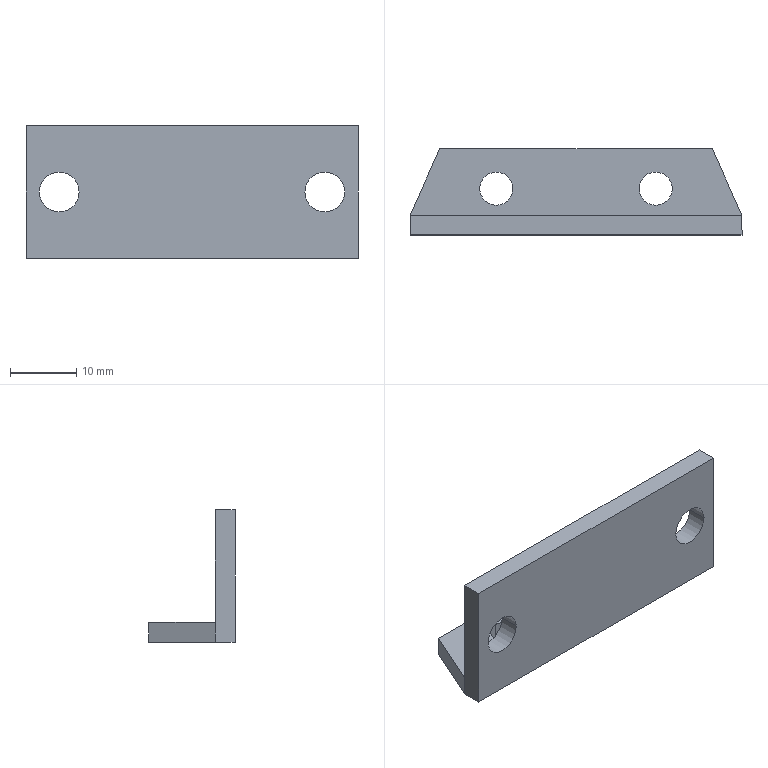Component | SolidWorks | Stand-2 | 1 solid | 18 faces | box 50 x 13 x 20 mm | volume 4078 mm3 | plane 10 | cylinder 8 | commonest cylinder face diameters 5 x4 6 x4
build123d program:
from build123d import *

# Parameters (mm, degrees)
SKETCH1_W      = 50
SKETCH1_H      = 20
SKETCH1_R      = 3
EXTRUDE1_DEPTH = 3
SKETCH2_R      = 2.5
EXTRUDE2_DEPTH = 3


with BuildPart() as part:
    # Sketch1 → Extrude1 (new body)
    with BuildSketch(Plane.XY):
        with Locations((-4.582, -13.446)):
            Rectangle(SKETCH1_W, SKETCH1_H)
        with Locations((-24.582, -13.446)):
            Circle(SKETCH1_R, mode=Mode.SUBTRACT)
        with Locations((15.418, -13.446)):
            Circle(SKETCH1_R, mode=Mode.SUBTRACT)
    extrude(amount=EXTRUDE1_DEPTH)

    # Sketch2 → Extrude2 (add)
    with BuildSketch(Plane.XZ.offset(23.446)):
        Polygon((-29.582, 3), (-25.108, 13), (15.944, 13), (20.418, 3), align=None)
        with Locations(Location((-16.582, 7, 0), (0, 0, 270))):
            Circle(SKETCH2_R, mode=Mode.SUBTRACT)
        with Locations(Location((7.418, 7, 0), (0, 0, 90))):
            Circle(SKETCH2_R, mode=Mode.SUBTRACT)
    extrude(amount=-EXTRUDE2_DEPTH)


solid = part.part

# Placed as in the assembly
solid = solid.moved(Location((1.543, -20.646, 12.946), (-90, 0, 180)))
STEP:
#1=COLOUR_RGB('',0.7922,0.8196,0.9333);
#2=FILL_AREA_STYLE_COLOUR('',#1);
#3=FILL_AREA_STYLE('',(#2));
#4=SURFACE_STYLE_FILL_AREA(#3);
#5=SURFACE_SIDE_STYLE('',(#4));
#6=SURFACE_STYLE_USAGE(.BOTH.,#5);
#7=PRESENTATION_STYLE_ASSIGNMENT((#6));
#8=CARTESIAN_POINT('',(-0.2313,-0.4388,-0.2953));
#9=VERTEX_POINT('',#8);
#10=CARTESIAN_POINT('',(-0.2313,-0.6357,-0.2953));
#11=VERTEX_POINT('',#10);
#12=CARTESIAN_POINT('',(-0.2313,-0.5373,-0.2953));
#13=DIRECTION('',(0.,0.,-1.));
#14=DIRECTION('',(-0.,1.,0.));
#15=AXIS2_PLACEMENT_3D('',#12,#13,#14);
#16=CIRCLE('',#15,0.09843);
#17=EDGE_CURVE('',#9,#11,#16,.T.);
#18=ORIENTED_EDGE('',*,*,#17,.F.);
#19=CARTESIAN_POINT('',(-0.2313,-0.4388,-0.4134));
#20=VERTEX_POINT('',#19);
#21=CARTESIAN_POINT('',(-0.2313,-0.4388,-0.2953));
#22=DIRECTION('',(0.,0.,-1.));
#23=VECTOR('',#22,39.37);
#24=LINE('',#21,#23);
#25=EDGE_CURVE('',#9,#20,#24,.T.);
#26=ORIENTED_EDGE('',*,*,#25,.T.);
#27=CARTESIAN_POINT('',(-0.2313,-0.6357,-0.4134));
#28=VERTEX_POINT('',#27);
#29=CARTESIAN_POINT('',(-0.2313,-0.5373,-0.4134));
#30=DIRECTION('',(0.,0.,-1.));
#31=DIRECTION('',(-0.,1.,0.));
#32=AXIS2_PLACEMENT_3D('',#29,#30,#31);
#33=CIRCLE('',#32,0.09843);
#34=EDGE_CURVE('',#20,#28,#33,.T.);
#35=ORIENTED_EDGE('',*,*,#34,.T.);
#36=CARTESIAN_POINT('',(-0.2313,-0.6357,-0.2953));
#37=DIRECTION('',(0.,0.,-1.));
#38=VECTOR('',#37,39.37);
#39=LINE('',#36,#38);
#40=EDGE_CURVE('',#11,#28,#39,.T.);
#41=ORIENTED_EDGE('',*,*,#40,.F.);
#42=EDGE_LOOP('',(#18,#26,#35,#41));
#43=FACE_OUTER_BOUND('',#42,.T.);
#44=CARTESIAN_POINT('',(-0.2313,-0.5373,-0.2953));
#45=DIRECTION('',(0.,0.,-1.));
#46=DIRECTION('',(0.,-1.,0.));
#47=AXIS2_PLACEMENT_3D('',#44,#45,#46);
#48=CYLINDRICAL_SURFACE('',#47,0.09843);
#49=ADVANCED_FACE('',(#43),#48,.F.);
#50=CARTESIAN_POINT('',(0.7136,-0.4388,-0.2953));
#51=VERTEX_POINT('',#50);
#52=CARTESIAN_POINT('',(0.7136,-0.6357,-0.2953));
#53=VERTEX_POINT('',#52);
#54=CARTESIAN_POINT('',(0.7136,-0.5373,-0.2953));
#55=DIRECTION('',(0.,0.,-1.));
#56=DIRECTION('',(0.,-1.,0.));
#57=AXIS2_PLACEMENT_3D('',#54,#55,#56);
#58=CIRCLE('',#57,0.09843);
#59=EDGE_CURVE('',#51,#53,#58,.T.);
#60=ORIENTED_EDGE('',*,*,#59,.F.);
#61=CARTESIAN_POINT('',(0.7136,-0.4388,-0.4134));
#62=VERTEX_POINT('',#61);
#63=CARTESIAN_POINT('',(0.7136,-0.4388,-0.2953));
#64=DIRECTION('',(0.,0.,-1.));
#65=VECTOR('',#64,39.37);
#66=LINE('',#63,#65);
#67=EDGE_CURVE('',#51,#62,#66,.T.);
#68=ORIENTED_EDGE('',*,*,#67,.T.);
#69=CARTESIAN_POINT('',(0.7136,-0.6357,-0.4134));
#70=VERTEX_POINT('',#69);
#71=CARTESIAN_POINT('',(0.7136,-0.5373,-0.4134));
#72=DIRECTION('',(0.,0.,-1.));
#73=DIRECTION('',(0.,-1.,0.));
#74=AXIS2_PLACEMENT_3D('',#71,#72,#73);
#75=CIRCLE('',#74,0.09843);
#76=EDGE_CURVE('',#62,#70,#75,.T.);
#77=ORIENTED_EDGE('',*,*,#76,.T.);
#78=CARTESIAN_POINT('',(0.7136,-0.6357,-0.2953));
#79=DIRECTION('',(0.,0.,-1.));
#80=VECTOR('',#79,39.37);
#81=LINE('',#78,#80);
#82=EDGE_CURVE('',#53,#70,#81,.T.);
#83=ORIENTED_EDGE('',*,*,#82,.F.);
#84=EDGE_LOOP('',(#60,#68,#77,#83));
#85=FACE_OUTER_BOUND('',#84,.T.);
#86=CARTESIAN_POINT('',(0.7136,-0.5373,-0.2953));
#87=DIRECTION('',(0.,0.,-1.));
#88=DIRECTION('',(0.,-1.,0.));
#89=AXIS2_PLACEMENT_3D('',#86,#87,#88);
#90=CYLINDRICAL_SURFACE('',#89,0.09843);
#91=ADVANCED_FACE('',(#85),#90,.F.);
#92=CARTESIAN_POINT('',(-0.4282,-0.6947,-0.01969));
#93=VERTEX_POINT('',#92);
#94=CARTESIAN_POINT('',(-0.6644,-0.6947,-0.01969));
#95=VERTEX_POINT('',#94);
#96=CARTESIAN_POINT('',(-0.5463,-0.6947,-0.01969));
#97=DIRECTION('',(-0.,1.,0.));
#98=DIRECTION('',(-1.,-0.,-0.));
#99=AXIS2_PLACEMENT_3D('',#96,#97,#98);
#100=CIRCLE('',#99,0.1181);
#101=EDGE_CURVE('',#93,#95,#100,.T.);
#102=ORIENTED_EDGE('',*,*,#101,.T.);
#103=CARTESIAN_POINT('',(-0.6644,-0.8129,-0.01969));
#104=VERTEX_POINT('',#103);
#105=CARTESIAN_POINT('',(-0.6644,-0.6947,-0.01969));
#106=DIRECTION('',(0.,-1.,-0.));
#107=VECTOR('',#106,39.37);
#108=LINE('',#105,#107);
#109=EDGE_CURVE('',#95,#104,#108,.T.);
#110=ORIENTED_EDGE('',*,*,#109,.T.);
#111=CARTESIAN_POINT('',(-0.4282,-0.8129,-0.01969));
#112=VERTEX_POINT('',#111);
#113=CARTESIAN_POINT('',(-0.5463,-0.8129,-0.01969));
#114=DIRECTION('',(-0.,1.,0.));
#115=DIRECTION('',(-1.,-0.,-0.));
#116=AXIS2_PLACEMENT_3D('',#113,#114,#115);
#117=CIRCLE('',#116,0.1181);
#118=EDGE_CURVE('',#112,#104,#117,.T.);
#119=ORIENTED_EDGE('',*,*,#118,.F.);
#120=CARTESIAN_POINT('',(-0.4282,-0.6947,-0.01969));
#121=DIRECTION('',(0.,-1.,-0.));
#122=VECTOR('',#121,39.37);
#123=LINE('',#120,#122);
#124=EDGE_CURVE('',#93,#112,#123,.T.);
#125=ORIENTED_EDGE('',*,*,#124,.F.);
#126=EDGE_LOOP('',(#102,#110,#119,#125));
#127=FACE_OUTER_BOUND('',#126,.T.);
#128=CARTESIAN_POINT('',(-0.5463,-0.6947,-0.01969));
#129=DIRECTION('',(0.,-1.,-0.));
#130=DIRECTION('',(1.,0.,0.));
#131=AXIS2_PLACEMENT_3D('',#128,#129,#130);
#132=CYLINDRICAL_SURFACE('',#131,0.1181);
#133=ADVANCED_FACE('',(#127),#132,.F.);
#134=CARTESIAN_POINT('',(1.147,-0.6947,-0.01969));
#135=VERTEX_POINT('',#134);
#136=CARTESIAN_POINT('',(0.9104,-0.6947,-0.01969));
#137=VERTEX_POINT('',#136);
#138=CARTESIAN_POINT('',(1.029,-0.6947,-0.01969));
#139=DIRECTION('',(-0.,1.,0.));
#140=DIRECTION('',(-1.,-0.,-0.));
#141=AXIS2_PLACEMENT_3D('',#138,#139,#140);
#142=CIRCLE('',#141,0.1181);
#143=EDGE_CURVE('',#135,#137,#142,.T.);
#144=ORIENTED_EDGE('',*,*,#143,.T.);
#145=CARTESIAN_POINT('',(0.9104,-0.8129,-0.01969));
#146=VERTEX_POINT('',#145);
#147=CARTESIAN_POINT('',(0.9104,-0.6947,-0.01969));
#148=DIRECTION('',(0.,-1.,-0.));
#149=VECTOR('',#148,39.37);
#150=LINE('',#147,#149);
#151=EDGE_CURVE('',#137,#146,#150,.T.);
#152=ORIENTED_EDGE('',*,*,#151,.T.);
#153=CARTESIAN_POINT('',(1.147,-0.8129,-0.01969));
#154=VERTEX_POINT('',#153);
#155=CARTESIAN_POINT('',(1.029,-0.8129,-0.01969));
#156=DIRECTION('',(-0.,1.,0.));
#157=DIRECTION('',(-1.,-0.,-0.));
#158=AXIS2_PLACEMENT_3D('',#155,#156,#157);
#159=CIRCLE('',#158,0.1181);
#160=EDGE_CURVE('',#154,#146,#159,.T.);
#161=ORIENTED_EDGE('',*,*,#160,.F.);
#162=CARTESIAN_POINT('',(1.147,-0.6947,-0.01969));
#163=DIRECTION('',(0.,-1.,-0.));
#164=VECTOR('',#163,39.37);
#165=LINE('',#162,#164);
#166=EDGE_CURVE('',#135,#154,#165,.T.);
#167=ORIENTED_EDGE('',*,*,#166,.F.);
#168=EDGE_LOOP('',(#144,#152,#161,#167));
#169=FACE_OUTER_BOUND('',#168,.T.);
#170=CARTESIAN_POINT('',(1.029,-0.6947,-0.01969));
#171=DIRECTION('',(0.,-1.,-0.));
#172=DIRECTION('',(1.,0.,0.));
#173=AXIS2_PLACEMENT_3D('',#170,#171,#172);
#174=CYLINDRICAL_SURFACE('',#173,0.1181);
#175=ADVANCED_FACE('',(#169),#174,.F.);
#176=ORIENTED_EDGE('',*,*,#101,.F.);
#177=CARTESIAN_POINT('',(-0.5463,-0.6947,-0.01969));
#178=DIRECTION('',(-0.,1.,0.));
#179=DIRECTION('',(-1.,-0.,-0.));
#180=AXIS2_PLACEMENT_3D('',#177,#178,#179);
#181=CIRCLE('',#180,0.1181);
#182=EDGE_CURVE('',#95,#93,#181,.T.);
#183=ORIENTED_EDGE('',*,*,#182,.F.);
#184=EDGE_LOOP('',(#176,#183));
#185=FACE_BOUND('',#184,.T.);
#186=ORIENTED_EDGE('',*,*,#143,.F.);
#187=CARTESIAN_POINT('',(1.029,-0.6947,-0.01969));
#188=DIRECTION('',(-0.,1.,0.));
#189=DIRECTION('',(-1.,-0.,-0.));
#190=AXIS2_PLACEMENT_3D('',#187,#188,#189);
#191=CIRCLE('',#190,0.1181);
#192=EDGE_CURVE('',#137,#135,#191,.T.);
#193=ORIENTED_EDGE('',*,*,#192,.F.);
#194=EDGE_LOOP('',(#186,#193));
#195=FACE_BOUND('',#194,.T.);
#196=CARTESIAN_POINT('',(1.225,-0.6947,0.374));
#197=VERTEX_POINT('',#196);
#198=CARTESIAN_POINT('',(1.225,-0.6947,-0.2953));
#199=VERTEX_POINT('',#198);
#200=CARTESIAN_POINT('',(1.225,-0.6947,0.374));
#201=DIRECTION('',(0.,0.,-1.));
#202=VECTOR('',#201,39.37);
#203=LINE('',#200,#202);
#204=EDGE_CURVE('',#197,#199,#203,.T.);
#205=ORIENTED_EDGE('',*,*,#204,.T.);
#206=CARTESIAN_POINT('',(-0.7431,-0.6947,-0.2953));
#207=VERTEX_POINT('',#206);
#208=CARTESIAN_POINT('',(1.225,-0.6947,-0.2953));
#209=DIRECTION('',(-1.,-0.,-0.));
#210=VECTOR('',#209,39.37);
#211=LINE('',#208,#210);
#212=EDGE_CURVE('',#199,#207,#211,.T.);
#213=ORIENTED_EDGE('',*,*,#212,.T.);
#214=CARTESIAN_POINT('',(-0.7431,-0.6947,0.374));
#215=VERTEX_POINT('',#214);
#216=CARTESIAN_POINT('',(-0.7431,-0.6947,0.374));
#217=DIRECTION('',(0.,-0.,1.));
#218=VECTOR('',#217,39.37);
#219=LINE('',#216,#218);
#220=EDGE_CURVE('',#207,#215,#219,.T.);
#221=ORIENTED_EDGE('',*,*,#220,.T.);
#222=CARTESIAN_POINT('',(1.225,-0.6947,0.374));
#223=DIRECTION('',(1.,0.,0.));
#224=VECTOR('',#223,39.37);
#225=LINE('',#222,#224);
#226=EDGE_CURVE('',#215,#197,#225,.T.);
#227=ORIENTED_EDGE('',*,*,#226,.T.);
#228=EDGE_LOOP('',(#205,#213,#221,#227));
#229=FACE_OUTER_BOUND('',#228,.T.);
#230=CARTESIAN_POINT('',(1.225,-0.6947,-0.4134));
#231=DIRECTION('',(-0.,1.,0.));
#232=DIRECTION('',(-1.,-0.,-0.));
#233=AXIS2_PLACEMENT_3D('',#230,#231,#232);
#234=PLANE('',#233);
#235=ADVANCED_FACE('',(#185,#195,#229),#234,.T.);
#236=ORIENTED_EDGE('',*,*,#160,.T.);
#237=CARTESIAN_POINT('',(1.029,-0.8129,-0.01969));
#238=DIRECTION('',(-0.,1.,0.));
#239=DIRECTION('',(-1.,-0.,-0.));
#240=AXIS2_PLACEMENT_3D('',#237,#238,#239);
#241=CIRCLE('',#240,0.1181);
#242=EDGE_CURVE('',#146,#154,#241,.T.);
#243=ORIENTED_EDGE('',*,*,#242,.T.);
#244=EDGE_LOOP('',(#236,#243));
#245=FACE_BOUND('',#244,.T.);
#246=CARTESIAN_POINT('',(1.225,-0.8129,0.374));
#247=VERTEX_POINT('',#246);
#248=CARTESIAN_POINT('',(1.225,-0.8129,-0.4134));
#249=VERTEX_POINT('',#248);
#250=CARTESIAN_POINT('',(1.225,-0.8129,0.374));
#251=DIRECTION('',(0.,0.,-1.));
#252=VECTOR('',#251,39.37);
#253=LINE('',#250,#252);
#254=EDGE_CURVE('',#247,#249,#253,.T.);
#255=ORIENTED_EDGE('',*,*,#254,.F.);
#256=CARTESIAN_POINT('',(-0.7431,-0.8129,0.374));
#257=VERTEX_POINT('',#256);
#258=CARTESIAN_POINT('',(1.225,-0.8129,0.374));
#259=DIRECTION('',(1.,0.,0.));
#260=VECTOR('',#259,39.37);
#261=LINE('',#258,#260);
#262=EDGE_CURVE('',#257,#247,#261,.T.);
#263=ORIENTED_EDGE('',*,*,#262,.F.);
#264=CARTESIAN_POINT('',(-0.7431,-0.8129,-0.4134));
#265=VERTEX_POINT('',#264);
#266=CARTESIAN_POINT('',(-0.7431,-0.8129,0.374));
#267=DIRECTION('',(0.,-0.,1.));
#268=VECTOR('',#267,39.37);
#269=LINE('',#266,#268);
#270=EDGE_CURVE('',#265,#257,#269,.T.);
#271=ORIENTED_EDGE('',*,*,#270,.F.);
#272=CARTESIAN_POINT('',(1.225,-0.8129,-0.4134));
#273=DIRECTION('',(-1.,-0.,-0.));
#274=VECTOR('',#273,39.37);
#275=LINE('',#272,#274);
#276=EDGE_CURVE('',#249,#265,#275,.T.);
#277=ORIENTED_EDGE('',*,*,#276,.F.);
#278=EDGE_LOOP('',(#255,#263,#271,#277));
#279=FACE_OUTER_BOUND('',#278,.T.);
#280=ORIENTED_EDGE('',*,*,#118,.T.);
#281=CARTESIAN_POINT('',(-0.5463,-0.8129,-0.01969));
#282=DIRECTION('',(-0.,1.,0.));
#283=DIRECTION('',(-1.,-0.,-0.));
#284=AXIS2_PLACEMENT_3D('',#281,#282,#283);
#285=CIRCLE('',#284,0.1181);
#286=EDGE_CURVE('',#104,#112,#285,.T.);
#287=ORIENTED_EDGE('',*,*,#286,.T.);
#288=EDGE_LOOP('',(#280,#287));
#289=FACE_BOUND('',#288,.T.);
#290=CARTESIAN_POINT('',(1.225,-0.8129,-0.4134));
#291=DIRECTION('',(-0.,1.,0.));
#292=DIRECTION('',(-1.,-0.,-0.));
#293=AXIS2_PLACEMENT_3D('',#290,#291,#292);
#294=PLANE('',#293);
#295=ADVANCED_FACE('',(#245,#279,#289),#294,.F.);
#296=ORIENTED_EDGE('',*,*,#254,.T.);
#297=CARTESIAN_POINT('',(1.225,-0.6947,-0.4134));
#298=VERTEX_POINT('',#297);
#299=CARTESIAN_POINT('',(1.225,-0.6947,-0.4134));
#300=DIRECTION('',(0.,-1.,-0.));
#301=VECTOR('',#300,39.37);
#302=LINE('',#299,#301);
#303=EDGE_CURVE('',#298,#249,#302,.T.);
#304=ORIENTED_EDGE('',*,*,#303,.F.);
#305=CARTESIAN_POINT('',(1.225,-0.6947,-0.2953));
#306=DIRECTION('',(0.,0.,-1.));
#307=VECTOR('',#306,39.37);
#308=LINE('',#305,#307);
#309=EDGE_CURVE('',#199,#298,#308,.T.);
#310=ORIENTED_EDGE('',*,*,#309,.F.);
#311=ORIENTED_EDGE('',*,*,#204,.F.);
#312=CARTESIAN_POINT('',(1.225,-0.6947,0.374));
#313=DIRECTION('',(0.,-1.,-0.));
#314=VECTOR('',#313,39.37);
#315=LINE('',#312,#314);
#316=EDGE_CURVE('',#197,#247,#315,.T.);
#317=ORIENTED_EDGE('',*,*,#316,.T.);
#318=EDGE_LOOP('',(#296,#304,#310,#311,#317));
#319=FACE_OUTER_BOUND('',#318,.T.);
#320=CARTESIAN_POINT('',(1.225,-0.6947,0.374));
#321=DIRECTION('',(-1.,-0.,-0.));
#322=DIRECTION('',(0.,-1.,-0.));
#323=AXIS2_PLACEMENT_3D('',#320,#321,#322);
#324=PLANE('',#323);
#325=ADVANCED_FACE('',(#319),#324,.F.);
#326=ORIENTED_EDGE('',*,*,#276,.T.);
#327=CARTESIAN_POINT('',(-0.7431,-0.6947,-0.4134));
#328=VERTEX_POINT('',#327);
#329=CARTESIAN_POINT('',(-0.7431,-0.6947,-0.4134));
#330=DIRECTION('',(0.,-1.,-0.));
#331=VECTOR('',#330,39.37);
#332=LINE('',#329,#331);
#333=EDGE_CURVE('',#328,#265,#332,.T.);
#334=ORIENTED_EDGE('',*,*,#333,.F.);
#335=CARTESIAN_POINT('',(-0.567,-0.301,-0.4134));
#336=VERTEX_POINT('',#335);
#337=CARTESIAN_POINT('',(-0.7431,-0.6947,-0.4134));
#338=DIRECTION('',(0.4084,0.9128,0.));
#339=VECTOR('',#338,39.37);
#340=LINE('',#337,#339);
#341=EDGE_CURVE('',#328,#336,#340,.T.);
#342=ORIENTED_EDGE('',*,*,#341,.T.);
#343=CARTESIAN_POINT('',(1.049,-0.301,-0.4134));
#344=VERTEX_POINT('',#343);
#345=CARTESIAN_POINT('',(1.049,-0.301,-0.4134));
#346=DIRECTION('',(1.,0.,0.));
#347=VECTOR('',#346,39.37);
#348=LINE('',#345,#347);
#349=EDGE_CURVE('',#336,#344,#348,.T.);
#350=ORIENTED_EDGE('',*,*,#349,.T.);
#351=CARTESIAN_POINT('',(1.225,-0.6947,-0.4134));
#352=DIRECTION('',(0.4084,-0.9128,-0.));
#353=VECTOR('',#352,39.37);
#354=LINE('',#351,#353);
#355=EDGE_CURVE('',#344,#298,#354,.T.);
#356=ORIENTED_EDGE('',*,*,#355,.T.);
#357=ORIENTED_EDGE('',*,*,#303,.T.);
#358=EDGE_LOOP('',(#326,#334,#342,#350,#356,#357));
#359=FACE_OUTER_BOUND('',#358,.T.);
#360=CARTESIAN_POINT('',(-0.2313,-0.5373,-0.4134));
#361=DIRECTION('',(0.,0.,-1.));
#362=DIRECTION('',(-0.,1.,0.));
#363=AXIS2_PLACEMENT_3D('',#360,#361,#362);
#364=CIRCLE('',#363,0.09843);
#365=EDGE_CURVE('',#28,#20,#364,.T.);
#366=ORIENTED_EDGE('',*,*,#365,.F.);
#367=ORIENTED_EDGE('',*,*,#34,.F.);
#368=EDGE_LOOP('',(#366,#367));
#369=FACE_BOUND('',#368,.T.);
#370=CARTESIAN_POINT('',(0.7136,-0.5373,-0.4134));
#371=DIRECTION('',(0.,0.,-1.));
#372=DIRECTION('',(0.,-1.,0.));
#373=AXIS2_PLACEMENT_3D('',#370,#371,#372);
#374=CIRCLE('',#373,0.09843);
#375=EDGE_CURVE('',#70,#62,#374,.T.);
#376=ORIENTED_EDGE('',*,*,#375,.F.);
#377=ORIENTED_EDGE('',*,*,#76,.F.);
#378=EDGE_LOOP('',(#376,#377));
#379=FACE_BOUND('',#378,.T.);
#380=CARTESIAN_POINT('',(1.225,-0.6947,-0.4134));
#381=DIRECTION('',(-0.,-0.,1.));
#382=DIRECTION('',(-0.,1.,0.));
#383=AXIS2_PLACEMENT_3D('',#380,#381,#382);
#384=PLANE('',#383);
#385=ADVANCED_FACE('',(#359,#369,#379),#384,.F.);
#386=ORIENTED_EDGE('',*,*,#270,.T.);
#387=CARTESIAN_POINT('',(-0.7431,-0.6947,0.374));
#388=DIRECTION('',(0.,-1.,-0.));
#389=VECTOR('',#388,39.37);
#390=LINE('',#387,#389);
#391=EDGE_CURVE('',#215,#257,#390,.T.);
#392=ORIENTED_EDGE('',*,*,#391,.F.);
#393=ORIENTED_EDGE('',*,*,#220,.F.);
#394=CARTESIAN_POINT('',(-0.7431,-0.6947,0.374));
#395=DIRECTION('',(0.,-0.,1.));
#396=VECTOR('',#395,39.37);
#397=LINE('',#394,#396);
#398=EDGE_CURVE('',#328,#207,#397,.T.);
#399=ORIENTED_EDGE('',*,*,#398,.F.);
#400=ORIENTED_EDGE('',*,*,#333,.T.);
#401=EDGE_LOOP('',(#386,#392,#393,#399,#400));
#402=FACE_OUTER_BOUND('',#401,.T.);
#403=CARTESIAN_POINT('',(-0.7431,-0.6947,0.374));
#404=DIRECTION('',(1.,0.,-0.));
#405=DIRECTION('',(-0.,0.,-1.));
#406=AXIS2_PLACEMENT_3D('',#403,#404,#405);
#407=PLANE('',#406);
#408=ADVANCED_FACE('',(#402),#407,.F.);
#409=ORIENTED_EDGE('',*,*,#262,.T.);
#410=ORIENTED_EDGE('',*,*,#316,.F.);
#411=ORIENTED_EDGE('',*,*,#226,.F.);
#412=ORIENTED_EDGE('',*,*,#391,.T.);
#413=EDGE_LOOP('',(#409,#410,#411,#412));
#414=FACE_OUTER_BOUND('',#413,.T.);
#415=CARTESIAN_POINT('',(1.225,-0.6947,0.374));
#416=DIRECTION('',(0.,0.,-1.));
#417=DIRECTION('',(0.,-1.,-0.));
#418=AXIS2_PLACEMENT_3D('',#415,#416,#417);
#419=PLANE('',#418);
#420=ADVANCED_FACE('',(#414),#419,.F.);
#421=ORIENTED_EDGE('',*,*,#151,.F.);
#422=ORIENTED_EDGE('',*,*,#192,.T.);
#423=ORIENTED_EDGE('',*,*,#166,.T.);
#424=ORIENTED_EDGE('',*,*,#242,.F.);
#425=EDGE_LOOP('',(#421,#422,#423,#424));
#426=FACE_OUTER_BOUND('',#425,.T.);
#427=CARTESIAN_POINT('',(1.029,-0.6947,-0.01969));
#428=DIRECTION('',(0.,-1.,-0.));
#429=DIRECTION('',(1.,0.,0.));
#430=AXIS2_PLACEMENT_3D('',#427,#428,#429);
#431=CYLINDRICAL_SURFACE('',#430,0.1181);
#432=ADVANCED_FACE('',(#426),#431,.F.);
#433=ORIENTED_EDGE('',*,*,#109,.F.);
#434=ORIENTED_EDGE('',*,*,#182,.T.);
#435=ORIENTED_EDGE('',*,*,#124,.T.);
#436=ORIENTED_EDGE('',*,*,#286,.F.);
#437=EDGE_LOOP('',(#433,#434,#435,#436));
#438=FACE_OUTER_BOUND('',#437,.T.);
#439=CARTESIAN_POINT('',(-0.5463,-0.6947,-0.01969));
#440=DIRECTION('',(0.,-1.,-0.));
#441=DIRECTION('',(1.,0.,0.));
#442=AXIS2_PLACEMENT_3D('',#439,#440,#441);
#443=CYLINDRICAL_SURFACE('',#442,0.1181);
#444=ADVANCED_FACE('',(#438),#443,.F.);
#445=ORIENTED_EDGE('',*,*,#355,.F.);
#446=CARTESIAN_POINT('',(1.049,-0.301,-0.2953));
#447=VERTEX_POINT('',#446);
#448=CARTESIAN_POINT('',(1.049,-0.301,-0.2953));
#449=DIRECTION('',(0.,0.,-1.));
#450=VECTOR('',#449,39.37);
#451=LINE('',#448,#450);
#452=EDGE_CURVE('',#447,#344,#451,.T.);
#453=ORIENTED_EDGE('',*,*,#452,.F.);
#454=CARTESIAN_POINT('',(1.225,-0.6947,-0.2953));
#455=DIRECTION('',(0.4084,-0.9128,-0.));
#456=VECTOR('',#455,39.37);
#457=LINE('',#454,#456);
#458=EDGE_CURVE('',#447,#199,#457,.T.);
#459=ORIENTED_EDGE('',*,*,#458,.T.);
#460=ORIENTED_EDGE('',*,*,#309,.T.);
#461=EDGE_LOOP('',(#445,#453,#459,#460));
#462=FACE_OUTER_BOUND('',#461,.T.);
#463=CARTESIAN_POINT('',(1.225,-0.6947,-0.2953));
#464=DIRECTION('',(0.9128,0.4084,0.));
#465=DIRECTION('',(-0.4084,0.9128,0.));
#466=AXIS2_PLACEMENT_3D('',#463,#464,#465);
#467=PLANE('',#466);
#468=ADVANCED_FACE('',(#462),#467,.T.);
#469=ORIENTED_EDGE('',*,*,#349,.F.);
#470=CARTESIAN_POINT('',(-0.567,-0.301,-0.2953));
#471=VERTEX_POINT('',#470);
#472=CARTESIAN_POINT('',(-0.567,-0.301,-0.2953));
#473=DIRECTION('',(0.,0.,-1.));
#474=VECTOR('',#473,39.37);
#475=LINE('',#472,#474);
#476=EDGE_CURVE('',#471,#336,#475,.T.);
#477=ORIENTED_EDGE('',*,*,#476,.F.);
#478=CARTESIAN_POINT('',(1.049,-0.301,-0.2953));
#479=DIRECTION('',(1.,0.,0.));
#480=VECTOR('',#479,39.37);
#481=LINE('',#478,#480);
#482=EDGE_CURVE('',#471,#447,#481,.T.);
#483=ORIENTED_EDGE('',*,*,#482,.T.);
#484=ORIENTED_EDGE('',*,*,#452,.T.);
#485=EDGE_LOOP('',(#469,#477,#483,#484));
#486=FACE_OUTER_BOUND('',#485,.T.);
#487=CARTESIAN_POINT('',(1.049,-0.301,-0.2953));
#488=DIRECTION('',(-0.,1.,0.));
#489=DIRECTION('',(-1.,-0.,-0.));
#490=AXIS2_PLACEMENT_3D('',#487,#488,#489);
#491=PLANE('',#490);
#492=ADVANCED_FACE('',(#486),#491,.T.);
#493=ORIENTED_EDGE('',*,*,#341,.F.);
#494=ORIENTED_EDGE('',*,*,#398,.T.);
#495=CARTESIAN_POINT('',(-0.7431,-0.6947,-0.2953));
#496=DIRECTION('',(0.4084,0.9128,0.));
#497=VECTOR('',#496,39.37);
#498=LINE('',#495,#497);
#499=EDGE_CURVE('',#207,#471,#498,.T.);
#500=ORIENTED_EDGE('',*,*,#499,.T.);
#501=ORIENTED_EDGE('',*,*,#476,.T.);
#502=EDGE_LOOP('',(#493,#494,#500,#501));
#503=FACE_OUTER_BOUND('',#502,.T.);
#504=CARTESIAN_POINT('',(-0.7431,-0.6947,-0.2953));
#505=DIRECTION('',(-0.9128,0.4084,-0.));
#506=DIRECTION('',(-0.4084,-0.9128,-0.));
#507=AXIS2_PLACEMENT_3D('',#504,#505,#506);
#508=PLANE('',#507);
#509=ADVANCED_FACE('',(#503),#508,.T.);
#510=CARTESIAN_POINT('',(-0.2313,-0.5373,-0.2953));
#511=DIRECTION('',(0.,0.,-1.));
#512=DIRECTION('',(-0.,1.,0.));
#513=AXIS2_PLACEMENT_3D('',#510,#511,#512);
#514=CIRCLE('',#513,0.09843);
#515=EDGE_CURVE('',#11,#9,#514,.T.);
#516=ORIENTED_EDGE('',*,*,#515,.T.);
#517=ORIENTED_EDGE('',*,*,#17,.T.);
#518=EDGE_LOOP('',(#516,#517));
#519=FACE_BOUND('',#518,.T.);
#520=CARTESIAN_POINT('',(0.7136,-0.5373,-0.2953));
#521=DIRECTION('',(0.,0.,-1.));
#522=DIRECTION('',(0.,-1.,0.));
#523=AXIS2_PLACEMENT_3D('',#520,#521,#522);
#524=CIRCLE('',#523,0.09843);
#525=EDGE_CURVE('',#53,#51,#524,.T.);
#526=ORIENTED_EDGE('',*,*,#525,.T.);
#527=ORIENTED_EDGE('',*,*,#59,.T.);
#528=EDGE_LOOP('',(#526,#527));
#529=FACE_BOUND('',#528,.T.);
#530=ORIENTED_EDGE('',*,*,#212,.F.);
#531=ORIENTED_EDGE('',*,*,#458,.F.);
#532=ORIENTED_EDGE('',*,*,#482,.F.);
#533=ORIENTED_EDGE('',*,*,#499,.F.);
#534=EDGE_LOOP('',(#530,#531,#532,#533));
#535=FACE_OUTER_BOUND('',#534,.T.);
#536=CARTESIAN_POINT('',(-0.7431,-0.6947,-0.2953));
#537=DIRECTION('',(0.,0.,-1.));
#538=DIRECTION('',(0.,-1.,-0.));
#539=AXIS2_PLACEMENT_3D('',#536,#537,#538);
#540=PLANE('',#539);
#541=ADVANCED_FACE('',(#519,#529,#535),#540,.F.);
#542=ORIENTED_EDGE('',*,*,#67,.F.);
#543=ORIENTED_EDGE('',*,*,#525,.F.);
#544=ORIENTED_EDGE('',*,*,#82,.T.);
#545=ORIENTED_EDGE('',*,*,#375,.T.);
#546=EDGE_LOOP('',(#542,#543,#544,#545));
#547=FACE_OUTER_BOUND('',#546,.T.);
#548=CARTESIAN_POINT('',(0.7136,-0.5373,-0.2953));
#549=DIRECTION('',(0.,0.,-1.));
#550=DIRECTION('',(0.,-1.,0.));
#551=AXIS2_PLACEMENT_3D('',#548,#549,#550);
#552=CYLINDRICAL_SURFACE('',#551,0.09843);
#553=ADVANCED_FACE('',(#547),#552,.F.);
#554=ORIENTED_EDGE('',*,*,#25,.F.);
#555=ORIENTED_EDGE('',*,*,#515,.F.);
#556=ORIENTED_EDGE('',*,*,#40,.T.);
#557=ORIENTED_EDGE('',*,*,#365,.T.);
#558=EDGE_LOOP('',(#554,#555,#556,#557));
#559=FACE_OUTER_BOUND('',#558,.T.);
#560=CARTESIAN_POINT('',(-0.2313,-0.5373,-0.2953));
#561=DIRECTION('',(0.,0.,-1.));
#562=DIRECTION('',(0.,-1.,0.));
#563=AXIS2_PLACEMENT_3D('',#560,#561,#562);
#564=CYLINDRICAL_SURFACE('',#563,0.09843);
#565=ADVANCED_FACE('',(#559),#564,.F.);
#566=CLOSED_SHELL('',(#49,#91,#133,#175,#235,#295,#325,#385,#408,#420,#432,#444,#468,#492,#509,#541,#553,#565));
#567=MANIFOLD_SOLID_BREP('',#566);
#568=STYLED_ITEM('',(#7),#567);
#569=(LENGTH_UNIT()NAMED_UNIT(*)SI_UNIT($,.METRE.));
#570=LENGTH_MEASURE_WITH_UNIT(LENGTH_MEASURE(0.0254),#569);
#571=DIMENSIONAL_EXPONENTS(1.,0.,0.,0.,0.,0.,0.);
#572=(CONVERSION_BASED_UNIT('',#570)LENGTH_UNIT()NAMED_UNIT(#571));
#573=UNCERTAINTY_MEASURE_WITH_UNIT(LENGTH_MEASURE(0.00001),#572,'','');
#574=(NAMED_UNIT(*)PLANE_ANGLE_UNIT()SI_UNIT($,.RADIAN.));
#575=(NAMED_UNIT(*)SI_UNIT($,.STERADIAN.)SOLID_ANGLE_UNIT());
#576=(GEOMETRIC_REPRESENTATION_CONTEXT(3)GLOBAL_UNCERTAINTY_ASSIGNED_CONTEXT((#573))GLOBAL_UNIT_ASSIGNED_CONTEXT((#572,#574,#575))REPRESENTATION_CONTEXT('',''));
#577=MECHANICAL_DESIGN_GEOMETRIC_PRESENTATION_REPRESENTATION('',(#568),#576);
#578=CARTESIAN_POINT('',(0.,0.,0.));
#579=DIRECTION('',(0.,0.,1.));
#580=DIRECTION('',(1.,0.,0.));
#581=AXIS2_PLACEMENT_3D('',#578,#579,#580);
#582=(LENGTH_UNIT()NAMED_UNIT(*)SI_UNIT($,.METRE.));
#583=LENGTH_MEASURE_WITH_UNIT(LENGTH_MEASURE(0.0254),#582);
#584=DIMENSIONAL_EXPONENTS(1.,0.,0.,0.,0.,0.,0.);
#585=(CONVERSION_BASED_UNIT('',#583)LENGTH_UNIT()NAMED_UNIT(#584));
#586=UNCERTAINTY_MEASURE_WITH_UNIT(LENGTH_MEASURE(0.00001),#585,'','');
#587=(NAMED_UNIT(*)PLANE_ANGLE_UNIT()SI_UNIT($,.RADIAN.));
#588=(NAMED_UNIT(*)SI_UNIT($,.STERADIAN.)SOLID_ANGLE_UNIT());
#589=(GEOMETRIC_REPRESENTATION_CONTEXT(3)GLOBAL_UNCERTAINTY_ASSIGNED_CONTEXT((#586))GLOBAL_UNIT_ASSIGNED_CONTEXT((#585,#587,#588))REPRESENTATION_CONTEXT('',''));
#590=ADVANCED_BREP_SHAPE_REPRESENTATION('',(#567,#581),#589);
#591=PRESENTATION_LAYER_ASSIGNMENT('','',(#568));